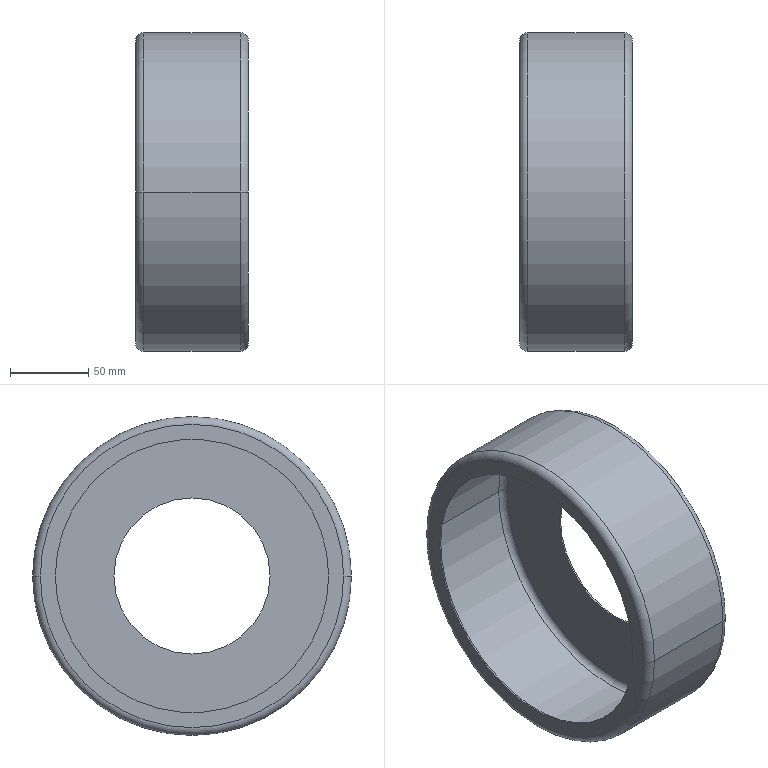Component | SolidWorks | Flywheel-1 | 1 solid | 20 faces | box 72.09 x 204.25 x 204.25 mm | volume 75898 mm3 | cylinder 8 | torus 8 | plane 4 | commonest cylinder face diameters 100 x2 204.252 x2 175 x2 202.252 x2
build123d program:
from build123d import *

# Parameters (mm, degrees)
SKETCH2_R                 = 50
REPAIR_CAMSHAFTHOLE_DEPTH = 1.75


with BuildPart() as part:
    # Sketch1 → Revolve1 (revolve)
    with BuildSketch(Plane(origin=(0, 0, 0), x_dir=(1, 0, 0), z_dir=(0, 1, 0))):
        with BuildLine():
            Line((97.126, 75), (0, 75))
            Line((0, 75), (0, 74))
            Line((0, 74), (97.126, 74))
            ThreePointArc((97.126, 74), (99.954, 72.828), (101.126, 70))
            Line((101.126, 70), (101.126, 7.905))
            ThreePointArc((101.126, 7.905), (99.954, 5.077), (97.126, 3.905))
            Line((97.126, 3.905), (87.5, 3.905))
            Line((87.5, 3.905), (87.5, 2.905))
            Line((87.5, 2.905), (97.126, 2.905))
            ThreePointArc((97.126, 2.905), (100.662, 4.37), (102.126, 7.905))
            Line((102.126, 7.905), (102.126, 70))
            ThreePointArc((102.126, 70), (100.662, 73.536), (97.126, 75))
        make_face()
    revolve(axis=Axis((0, 0, -75.001), (0, 0, 1)))

    # Sketch2 → Repair_CamshaftHole (cut, symmetric)
    with BuildSketch(Plane.XY.offset(-74.457)):
        Circle(SKETCH2_R)
    extrude(amount=REPAIR_CAMSHAFTHOLE_DEPTH, both=True, mode=Mode.SUBTRACT)


solid = part.part

# Placed as in the assembly
solid = solid.moved(Location((-829.707, 870.769, 1116.347), (0, -90, 0)))
STEP:
#1=CARTESIAN_POINT('',(-29.713,36.251,43.951));
#2=VERTEX_POINT('',#1);
#3=CARTESIAN_POINT('',(-29.713,32.314,43.951));
#4=VERTEX_POINT('',#3);
#5=CARTESIAN_POINT('',(-29.713,34.282,43.951));
#6=DIRECTION('',(1.,0.,0.));
#7=DIRECTION('',(0.,-1.,0.));
#8=AXIS2_PLACEMENT_3D('',#5,#6,#7);
#9=CIRCLE('',#8,1.969);
#10=EDGE_CURVE('',#2,#4,#9,.T.);
#11=ORIENTED_EDGE('',*,*,#10,.T.);
#12=CARTESIAN_POINT('',(-29.752,32.314,43.951));
#13=VERTEX_POINT('',#12);
#14=CARTESIAN_POINT('',(-29.665,32.314,43.951));
#15=DIRECTION('',(-1.,0.,0.));
#16=VECTOR('',#15,39.37);
#17=LINE('',#14,#16);
#18=EDGE_CURVE('',#4,#13,#17,.T.);
#19=ORIENTED_EDGE('',*,*,#18,.T.);
#20=CARTESIAN_POINT('',(-29.752,36.251,43.951));
#21=VERTEX_POINT('',#20);
#22=CARTESIAN_POINT('',(-29.752,34.282,43.951));
#23=DIRECTION('',(-1.,0.,0.));
#24=DIRECTION('',(0.,1.,0.));
#25=AXIS2_PLACEMENT_3D('',#22,#23,#24);
#26=CIRCLE('',#25,1.969);
#27=EDGE_CURVE('',#13,#21,#26,.T.);
#28=ORIENTED_EDGE('',*,*,#27,.T.);
#29=CARTESIAN_POINT('',(-29.665,36.251,43.951));
#30=DIRECTION('',(-1.,0.,0.));
#31=VECTOR('',#30,39.37);
#32=LINE('',#29,#31);
#33=EDGE_CURVE('',#2,#21,#32,.T.);
#34=ORIENTED_EDGE('',*,*,#33,.F.);
#35=EDGE_LOOP('',(#11,#19,#28,#34));
#36=FACE_OUTER_BOUND('',#35,.T.);
#37=CARTESIAN_POINT('',(-29.665,34.282,43.951));
#38=DIRECTION('',(-1.,0.,0.));
#39=DIRECTION('',(0.,1.,0.));
#40=AXIS2_PLACEMENT_3D('',#37,#38,#39);
#41=CYLINDRICAL_SURFACE('',#40,1.969);
#42=ADVANCED_FACE('',(#36),#41,.F.);
#43=CARTESIAN_POINT('',(-29.91,38.303,43.951));
#44=VERTEX_POINT('',#43);
#45=CARTESIAN_POINT('',(-29.91,30.262,43.951));
#46=VERTEX_POINT('',#45);
#47=CARTESIAN_POINT('',(-29.91,34.282,43.951));
#48=DIRECTION('',(-1.,0.,0.));
#49=DIRECTION('',(0.,1.,0.));
#50=AXIS2_PLACEMENT_3D('',#47,#48,#49);
#51=CIRCLE('',#50,4.021);
#52=EDGE_CURVE('',#44,#46,#51,.T.);
#53=ORIENTED_EDGE('',*,*,#52,.T.);
#54=CARTESIAN_POINT('',(-32.354,30.262,43.951));
#55=VERTEX_POINT('',#54);
#56=CARTESIAN_POINT('',(-29.713,30.262,43.951));
#57=DIRECTION('',(-1.,0.,0.));
#58=VECTOR('',#57,39.37);
#59=LINE('',#56,#58);
#60=EDGE_CURVE('',#46,#55,#59,.T.);
#61=ORIENTED_EDGE('',*,*,#60,.T.);
#62=CARTESIAN_POINT('',(-32.354,38.303,43.951));
#63=VERTEX_POINT('',#62);
#64=CARTESIAN_POINT('',(-32.354,34.282,43.951));
#65=DIRECTION('',(-1.,0.,0.));
#66=DIRECTION('',(0.,1.,0.));
#67=AXIS2_PLACEMENT_3D('',#64,#65,#66);
#68=CIRCLE('',#67,4.021);
#69=EDGE_CURVE('',#63,#55,#68,.T.);
#70=ORIENTED_EDGE('',*,*,#69,.F.);
#71=CARTESIAN_POINT('',(-29.713,38.303,43.951));
#72=DIRECTION('',(-1.,0.,0.));
#73=VECTOR('',#72,39.37);
#74=LINE('',#71,#73);
#75=EDGE_CURVE('',#44,#63,#74,.T.);
#76=ORIENTED_EDGE('',*,*,#75,.F.);
#77=EDGE_LOOP('',(#53,#61,#70,#76));
#78=FACE_OUTER_BOUND('',#77,.T.);
#79=CARTESIAN_POINT('',(-29.713,34.282,43.951));
#80=DIRECTION('',(-1.,0.,0.));
#81=DIRECTION('',(0.,1.,0.));
#82=AXIS2_PLACEMENT_3D('',#79,#80,#81);
#83=CYLINDRICAL_SURFACE('',#82,4.021);
#84=ADVANCED_FACE('',(#78),#83,.T.);
#85=ORIENTED_EDGE('',*,*,#69,.T.);
#86=CARTESIAN_POINT('',(-32.551,30.458,43.951));
#87=VERTEX_POINT('',#86);
#88=CARTESIAN_POINT('',(-32.354,30.458,43.951));
#89=DIRECTION('',(0.,0.,-1.));
#90=DIRECTION('',(0.,1.,0.));
#91=AXIS2_PLACEMENT_3D('',#88,#89,#90);
#92=CIRCLE('',#91,0.1969);
#93=EDGE_CURVE('',#55,#87,#92,.T.);
#94=ORIENTED_EDGE('',*,*,#93,.T.);
#95=CARTESIAN_POINT('',(-32.551,38.106,43.951));
#96=VERTEX_POINT('',#95);
#97=CARTESIAN_POINT('',(-32.551,34.282,43.951));
#98=DIRECTION('',(-1.,0.,0.));
#99=DIRECTION('',(0.,1.,0.));
#100=AXIS2_PLACEMENT_3D('',#97,#98,#99);
#101=CIRCLE('',#100,3.824);
#102=EDGE_CURVE('',#96,#87,#101,.T.);
#103=ORIENTED_EDGE('',*,*,#102,.F.);
#104=CARTESIAN_POINT('',(-32.354,38.106,43.951));
#105=DIRECTION('',(0.,0.,1.));
#106=DIRECTION('',(1.,0.,0.));
#107=AXIS2_PLACEMENT_3D('',#104,#105,#106);
#108=CIRCLE('',#107,0.1969);
#109=EDGE_CURVE('',#63,#96,#108,.T.);
#110=ORIENTED_EDGE('',*,*,#109,.F.);
#111=EDGE_LOOP('',(#85,#94,#103,#110));
#112=FACE_OUTER_BOUND('',#111,.T.);
#113=CARTESIAN_POINT('',(-32.354,34.282,43.951));
#114=DIRECTION('',(-1.,0.,0.));
#115=DIRECTION('',(0.,1.,0.));
#116=AXIS2_PLACEMENT_3D('',#113,#114,#115);
#117=TOROIDAL_SURFACE('',#116,3.824,0.1969);
#118=ADVANCED_FACE('',(#112),#117,.T.);
#119=CARTESIAN_POINT('',(-32.512,30.837,43.951));
#120=VERTEX_POINT('',#119);
#121=CARTESIAN_POINT('',(-32.512,37.727,43.951));
#122=VERTEX_POINT('',#121);
#123=CARTESIAN_POINT('',(-32.512,34.282,43.951));
#124=DIRECTION('',(-1.,0.,0.));
#125=DIRECTION('',(0.,1.,0.));
#126=AXIS2_PLACEMENT_3D('',#123,#124,#125);
#127=CIRCLE('',#126,3.445);
#128=EDGE_CURVE('',#120,#122,#127,.T.);
#129=ORIENTED_EDGE('',*,*,#128,.F.);
#130=CARTESIAN_POINT('',(-32.551,30.837,43.951));
#131=VERTEX_POINT('',#130);
#132=CARTESIAN_POINT('',(-29.713,30.837,43.951));
#133=DIRECTION('',(-1.,0.,0.));
#134=VECTOR('',#133,39.37);
#135=LINE('',#132,#134);
#136=EDGE_CURVE('',#120,#131,#135,.T.);
#137=ORIENTED_EDGE('',*,*,#136,.T.);
#138=CARTESIAN_POINT('',(-32.551,37.727,43.951));
#139=VERTEX_POINT('',#138);
#140=CARTESIAN_POINT('',(-32.551,34.282,43.951));
#141=DIRECTION('',(-1.,0.,0.));
#142=DIRECTION('',(0.,1.,0.));
#143=AXIS2_PLACEMENT_3D('',#140,#141,#142);
#144=CIRCLE('',#143,3.445);
#145=EDGE_CURVE('',#131,#139,#144,.T.);
#146=ORIENTED_EDGE('',*,*,#145,.T.);
#147=CARTESIAN_POINT('',(-29.713,37.727,43.951));
#148=DIRECTION('',(-1.,0.,0.));
#149=VECTOR('',#148,39.37);
#150=LINE('',#147,#149);
#151=EDGE_CURVE('',#122,#139,#150,.T.);
#152=ORIENTED_EDGE('',*,*,#151,.F.);
#153=EDGE_LOOP('',(#129,#137,#146,#152));
#154=FACE_OUTER_BOUND('',#153,.T.);
#155=CARTESIAN_POINT('',(-29.713,34.282,43.951));
#156=DIRECTION('',(-1.,0.,0.));
#157=DIRECTION('',(0.,1.,0.));
#158=AXIS2_PLACEMENT_3D('',#155,#156,#157);
#159=CYLINDRICAL_SURFACE('',#158,3.445);
#160=ADVANCED_FACE('',(#154),#159,.F.);
#161=CARTESIAN_POINT('',(-32.354,30.301,43.951));
#162=VERTEX_POINT('',#161);
#163=CARTESIAN_POINT('',(-32.354,38.264,43.951));
#164=VERTEX_POINT('',#163);
#165=CARTESIAN_POINT('',(-32.354,34.282,43.951));
#166=DIRECTION('',(-1.,0.,0.));
#167=DIRECTION('',(0.,1.,0.));
#168=AXIS2_PLACEMENT_3D('',#165,#166,#167);
#169=CIRCLE('',#168,3.981);
#170=EDGE_CURVE('',#162,#164,#169,.T.);
#171=ORIENTED_EDGE('',*,*,#170,.F.);
#172=CARTESIAN_POINT('',(-32.512,30.458,43.951));
#173=VERTEX_POINT('',#172);
#174=CARTESIAN_POINT('',(-32.354,30.458,43.951));
#175=DIRECTION('',(0.,0.,-1.));
#176=DIRECTION('',(0.,1.,0.));
#177=AXIS2_PLACEMENT_3D('',#174,#175,#176);
#178=CIRCLE('',#177,0.1575);
#179=EDGE_CURVE('',#162,#173,#178,.T.);
#180=ORIENTED_EDGE('',*,*,#179,.T.);
#181=CARTESIAN_POINT('',(-32.512,38.106,43.951));
#182=VERTEX_POINT('',#181);
#183=CARTESIAN_POINT('',(-32.512,34.282,43.951));
#184=DIRECTION('',(-1.,0.,0.));
#185=DIRECTION('',(0.,1.,0.));
#186=AXIS2_PLACEMENT_3D('',#183,#184,#185);
#187=CIRCLE('',#186,3.824);
#188=EDGE_CURVE('',#173,#182,#187,.T.);
#189=ORIENTED_EDGE('',*,*,#188,.T.);
#190=CARTESIAN_POINT('',(-32.354,38.106,43.951));
#191=DIRECTION('',(0.,0.,1.));
#192=DIRECTION('',(1.,0.,0.));
#193=AXIS2_PLACEMENT_3D('',#190,#191,#192);
#194=CIRCLE('',#193,0.1575);
#195=EDGE_CURVE('',#164,#182,#194,.T.);
#196=ORIENTED_EDGE('',*,*,#195,.F.);
#197=EDGE_LOOP('',(#171,#180,#189,#196));
#198=FACE_OUTER_BOUND('',#197,.T.);
#199=CARTESIAN_POINT('',(-32.354,34.282,43.951));
#200=DIRECTION('',(-1.,0.,0.));
#201=DIRECTION('',(0.,1.,0.));
#202=AXIS2_PLACEMENT_3D('',#199,#200,#201);
#203=TOROIDAL_SURFACE('',#202,3.824,0.1575);
#204=ADVANCED_FACE('',(#198),#203,.F.);
#205=CARTESIAN_POINT('',(-29.91,30.301,43.951));
#206=VERTEX_POINT('',#205);
#207=CARTESIAN_POINT('',(-29.91,38.264,43.951));
#208=VERTEX_POINT('',#207);
#209=CARTESIAN_POINT('',(-29.91,34.282,43.951));
#210=DIRECTION('',(-1.,0.,0.));
#211=DIRECTION('',(0.,1.,0.));
#212=AXIS2_PLACEMENT_3D('',#209,#210,#211);
#213=CIRCLE('',#212,3.981);
#214=EDGE_CURVE('',#206,#208,#213,.T.);
#215=ORIENTED_EDGE('',*,*,#214,.F.);
#216=CARTESIAN_POINT('',(-29.713,30.301,43.951));
#217=DIRECTION('',(-1.,0.,0.));
#218=VECTOR('',#217,39.37);
#219=LINE('',#216,#218);
#220=EDGE_CURVE('',#206,#162,#219,.T.);
#221=ORIENTED_EDGE('',*,*,#220,.T.);
#222=ORIENTED_EDGE('',*,*,#170,.T.);
#223=CARTESIAN_POINT('',(-29.713,38.264,43.951));
#224=DIRECTION('',(-1.,0.,0.));
#225=VECTOR('',#224,39.37);
#226=LINE('',#223,#225);
#227=EDGE_CURVE('',#208,#164,#226,.T.);
#228=ORIENTED_EDGE('',*,*,#227,.F.);
#229=EDGE_LOOP('',(#215,#221,#222,#228));
#230=FACE_OUTER_BOUND('',#229,.T.);
#231=CARTESIAN_POINT('',(-29.713,34.282,43.951));
#232=DIRECTION('',(-1.,0.,0.));
#233=DIRECTION('',(0.,1.,0.));
#234=AXIS2_PLACEMENT_3D('',#231,#232,#233);
#235=CYLINDRICAL_SURFACE('',#234,3.981);
#236=ADVANCED_FACE('',(#230),#235,.F.);
#237=CARTESIAN_POINT('',(-29.752,30.458,43.951));
#238=VERTEX_POINT('',#237);
#239=CARTESIAN_POINT('',(-29.752,38.106,43.951));
#240=VERTEX_POINT('',#239);
#241=CARTESIAN_POINT('',(-29.752,34.282,43.951));
#242=DIRECTION('',(-1.,0.,0.));
#243=DIRECTION('',(0.,1.,0.));
#244=AXIS2_PLACEMENT_3D('',#241,#242,#243);
#245=CIRCLE('',#244,3.824);
#246=EDGE_CURVE('',#238,#240,#245,.T.);
#247=ORIENTED_EDGE('',*,*,#246,.F.);
#248=CARTESIAN_POINT('',(-29.91,30.458,43.951));
#249=DIRECTION('',(0.,0.,-1.));
#250=DIRECTION('',(0.,1.,0.));
#251=AXIS2_PLACEMENT_3D('',#248,#249,#250);
#252=CIRCLE('',#251,0.1575);
#253=EDGE_CURVE('',#238,#206,#252,.T.);
#254=ORIENTED_EDGE('',*,*,#253,.T.);
#255=ORIENTED_EDGE('',*,*,#214,.T.);
#256=CARTESIAN_POINT('',(-29.91,38.106,43.951));
#257=DIRECTION('',(0.,0.,1.));
#258=DIRECTION('',(1.,0.,0.));
#259=AXIS2_PLACEMENT_3D('',#256,#257,#258);
#260=CIRCLE('',#259,0.1575);
#261=EDGE_CURVE('',#240,#208,#260,.T.);
#262=ORIENTED_EDGE('',*,*,#261,.F.);
#263=EDGE_LOOP('',(#247,#254,#255,#262));
#264=FACE_OUTER_BOUND('',#263,.T.);
#265=CARTESIAN_POINT('',(-29.91,34.282,43.951));
#266=DIRECTION('',(-1.,0.,0.));
#267=DIRECTION('',(0.,1.,0.));
#268=AXIS2_PLACEMENT_3D('',#265,#266,#267);
#269=TOROIDAL_SURFACE('',#268,3.824,0.1575);
#270=ADVANCED_FACE('',(#264),#269,.F.);
#271=CARTESIAN_POINT('',(-29.713,38.106,43.951));
#272=VERTEX_POINT('',#271);
#273=CARTESIAN_POINT('',(-29.713,30.458,43.951));
#274=VERTEX_POINT('',#273);
#275=CARTESIAN_POINT('',(-29.713,34.282,43.951));
#276=DIRECTION('',(-1.,0.,0.));
#277=DIRECTION('',(0.,1.,0.));
#278=AXIS2_PLACEMENT_3D('',#275,#276,#277);
#279=CIRCLE('',#278,3.824);
#280=EDGE_CURVE('',#272,#274,#279,.T.);
#281=ORIENTED_EDGE('',*,*,#280,.T.);
#282=CARTESIAN_POINT('',(-29.91,30.458,43.951));
#283=DIRECTION('',(0.,0.,-1.));
#284=DIRECTION('',(0.,1.,0.));
#285=AXIS2_PLACEMENT_3D('',#282,#283,#284);
#286=CIRCLE('',#285,0.1969);
#287=EDGE_CURVE('',#274,#46,#286,.T.);
#288=ORIENTED_EDGE('',*,*,#287,.T.);
#289=ORIENTED_EDGE('',*,*,#52,.F.);
#290=CARTESIAN_POINT('',(-29.91,38.106,43.951));
#291=DIRECTION('',(0.,0.,1.));
#292=DIRECTION('',(1.,0.,0.));
#293=AXIS2_PLACEMENT_3D('',#290,#291,#292);
#294=CIRCLE('',#293,0.1969);
#295=EDGE_CURVE('',#272,#44,#294,.T.);
#296=ORIENTED_EDGE('',*,*,#295,.F.);
#297=EDGE_LOOP('',(#281,#288,#289,#296));
#298=FACE_OUTER_BOUND('',#297,.T.);
#299=CARTESIAN_POINT('',(-29.91,34.282,43.951));
#300=DIRECTION('',(-1.,0.,0.));
#301=DIRECTION('',(0.,1.,0.));
#302=AXIS2_PLACEMENT_3D('',#299,#300,#301);
#303=TOROIDAL_SURFACE('',#302,3.824,0.1969);
#304=ADVANCED_FACE('',(#298),#303,.T.);
#305=ORIENTED_EDGE('',*,*,#287,.F.);
#306=CARTESIAN_POINT('',(-29.713,34.282,43.951));
#307=DIRECTION('',(-1.,0.,0.));
#308=DIRECTION('',(0.,1.,0.));
#309=AXIS2_PLACEMENT_3D('',#306,#307,#308);
#310=CIRCLE('',#309,3.824);
#311=EDGE_CURVE('',#274,#272,#310,.T.);
#312=ORIENTED_EDGE('',*,*,#311,.T.);
#313=ORIENTED_EDGE('',*,*,#295,.T.);
#314=CARTESIAN_POINT('',(-29.91,34.282,43.951));
#315=DIRECTION('',(-1.,0.,0.));
#316=DIRECTION('',(0.,1.,0.));
#317=AXIS2_PLACEMENT_3D('',#314,#315,#316);
#318=CIRCLE('',#317,4.021);
#319=EDGE_CURVE('',#46,#44,#318,.T.);
#320=ORIENTED_EDGE('',*,*,#319,.F.);
#321=EDGE_LOOP('',(#305,#312,#313,#320));
#322=FACE_OUTER_BOUND('',#321,.T.);
#323=CARTESIAN_POINT('',(-29.91,34.282,43.951));
#324=DIRECTION('',(-1.,0.,0.));
#325=DIRECTION('',(0.,1.,0.));
#326=AXIS2_PLACEMENT_3D('',#323,#324,#325);
#327=TOROIDAL_SURFACE('',#326,3.824,0.1969);
#328=ADVANCED_FACE('',(#322),#327,.T.);
#329=ORIENTED_EDGE('',*,*,#10,.F.);
#330=CARTESIAN_POINT('',(-29.713,34.282,43.951));
#331=DIRECTION('',(1.,0.,0.));
#332=DIRECTION('',(0.,-1.,0.));
#333=AXIS2_PLACEMENT_3D('',#330,#331,#332);
#334=CIRCLE('',#333,1.969);
#335=EDGE_CURVE('',#4,#2,#334,.T.);
#336=ORIENTED_EDGE('',*,*,#335,.F.);
#337=EDGE_LOOP('',(#329,#336));
#338=FACE_BOUND('',#337,.T.);
#339=ORIENTED_EDGE('',*,*,#280,.F.);
#340=ORIENTED_EDGE('',*,*,#311,.F.);
#341=EDGE_LOOP('',(#339,#340));
#342=FACE_OUTER_BOUND('',#341,.T.);
#343=CARTESIAN_POINT('',(-29.713,38.106,43.951));
#344=DIRECTION('',(1.,0.,0.));
#345=DIRECTION('',(0.,-1.,0.));
#346=AXIS2_PLACEMENT_3D('',#343,#344,#345);
#347=PLANE('',#346);
#348=ADVANCED_FACE('',(#338,#342),#347,.T.);
#349=CARTESIAN_POINT('',(-29.752,34.282,43.951));
#350=DIRECTION('',(-1.,0.,0.));
#351=DIRECTION('',(0.,1.,0.));
#352=AXIS2_PLACEMENT_3D('',#349,#350,#351);
#353=CIRCLE('',#352,1.969);
#354=EDGE_CURVE('',#21,#13,#353,.T.);
#355=ORIENTED_EDGE('',*,*,#354,.F.);
#356=ORIENTED_EDGE('',*,*,#27,.F.);
#357=EDGE_LOOP('',(#355,#356));
#358=FACE_BOUND('',#357,.T.);
#359=CARTESIAN_POINT('',(-29.752,34.282,43.951));
#360=DIRECTION('',(-1.,0.,0.));
#361=DIRECTION('',(0.,1.,0.));
#362=AXIS2_PLACEMENT_3D('',#359,#360,#361);
#363=CIRCLE('',#362,3.824);
#364=EDGE_CURVE('',#240,#238,#363,.T.);
#365=ORIENTED_EDGE('',*,*,#364,.T.);
#366=ORIENTED_EDGE('',*,*,#246,.T.);
#367=EDGE_LOOP('',(#365,#366));
#368=FACE_OUTER_BOUND('',#367,.T.);
#369=CARTESIAN_POINT('',(-29.752,34.282,43.951));
#370=DIRECTION('',(-1.,0.,0.));
#371=DIRECTION('',(0.,1.,0.));
#372=AXIS2_PLACEMENT_3D('',#369,#370,#371);
#373=PLANE('',#372);
#374=ADVANCED_FACE('',(#358,#368),#373,.T.);
#375=ORIENTED_EDGE('',*,*,#253,.F.);
#376=ORIENTED_EDGE('',*,*,#364,.F.);
#377=ORIENTED_EDGE('',*,*,#261,.T.);
#378=CARTESIAN_POINT('',(-29.91,34.282,43.951));
#379=DIRECTION('',(-1.,0.,0.));
#380=DIRECTION('',(0.,1.,0.));
#381=AXIS2_PLACEMENT_3D('',#378,#379,#380);
#382=CIRCLE('',#381,3.981);
#383=EDGE_CURVE('',#208,#206,#382,.T.);
#384=ORIENTED_EDGE('',*,*,#383,.T.);
#385=EDGE_LOOP('',(#375,#376,#377,#384));
#386=FACE_OUTER_BOUND('',#385,.T.);
#387=CARTESIAN_POINT('',(-29.91,34.282,43.951));
#388=DIRECTION('',(-1.,0.,0.));
#389=DIRECTION('',(0.,1.,0.));
#390=AXIS2_PLACEMENT_3D('',#387,#388,#389);
#391=TOROIDAL_SURFACE('',#390,3.824,0.1575);
#392=ADVANCED_FACE('',(#386),#391,.F.);
#393=ORIENTED_EDGE('',*,*,#220,.F.);
#394=ORIENTED_EDGE('',*,*,#383,.F.);
#395=ORIENTED_EDGE('',*,*,#227,.T.);
#396=CARTESIAN_POINT('',(-32.354,34.282,43.951));
#397=DIRECTION('',(-1.,0.,0.));
#398=DIRECTION('',(0.,1.,0.));
#399=AXIS2_PLACEMENT_3D('',#396,#397,#398);
#400=CIRCLE('',#399,3.981);
#401=EDGE_CURVE('',#164,#162,#400,.T.);
#402=ORIENTED_EDGE('',*,*,#401,.T.);
#403=EDGE_LOOP('',(#393,#394,#395,#402));
#404=FACE_OUTER_BOUND('',#403,.T.);
#405=CARTESIAN_POINT('',(-29.713,34.282,43.951));
#406=DIRECTION('',(-1.,0.,0.));
#407=DIRECTION('',(0.,1.,0.));
#408=AXIS2_PLACEMENT_3D('',#405,#406,#407);
#409=CYLINDRICAL_SURFACE('',#408,3.981);
#410=ADVANCED_FACE('',(#404),#409,.F.);
#411=ORIENTED_EDGE('',*,*,#179,.F.);
#412=ORIENTED_EDGE('',*,*,#401,.F.);
#413=ORIENTED_EDGE('',*,*,#195,.T.);
#414=CARTESIAN_POINT('',(-32.512,34.282,43.951));
#415=DIRECTION('',(-1.,0.,0.));
#416=DIRECTION('',(0.,1.,0.));
#417=AXIS2_PLACEMENT_3D('',#414,#415,#416);
#418=CIRCLE('',#417,3.824);
#419=EDGE_CURVE('',#182,#173,#418,.T.);
#420=ORIENTED_EDGE('',*,*,#419,.T.);
#421=EDGE_LOOP('',(#411,#412,#413,#420));
#422=FACE_OUTER_BOUND('',#421,.T.);
#423=CARTESIAN_POINT('',(-32.354,34.282,43.951));
#424=DIRECTION('',(-1.,0.,0.));
#425=DIRECTION('',(0.,1.,0.));
#426=AXIS2_PLACEMENT_3D('',#423,#424,#425);
#427=TOROIDAL_SURFACE('',#426,3.824,0.1575);
#428=ADVANCED_FACE('',(#422),#427,.F.);
#429=CARTESIAN_POINT('',(-32.512,34.282,43.951));
#430=DIRECTION('',(-1.,0.,0.));
#431=DIRECTION('',(0.,1.,0.));
#432=AXIS2_PLACEMENT_3D('',#429,#430,#431);
#433=CIRCLE('',#432,3.445);
#434=EDGE_CURVE('',#122,#120,#433,.T.);
#435=ORIENTED_EDGE('',*,*,#434,.T.);
#436=ORIENTED_EDGE('',*,*,#128,.T.);
#437=EDGE_LOOP('',(#435,#436));
#438=FACE_BOUND('',#437,.T.);
#439=ORIENTED_EDGE('',*,*,#419,.F.);
#440=ORIENTED_EDGE('',*,*,#188,.F.);
#441=EDGE_LOOP('',(#439,#440));
#442=FACE_OUTER_BOUND('',#441,.T.);
#443=CARTESIAN_POINT('',(-32.512,38.106,43.951));
#444=DIRECTION('',(1.,0.,0.));
#445=DIRECTION('',(0.,-1.,0.));
#446=AXIS2_PLACEMENT_3D('',#443,#444,#445);
#447=PLANE('',#446);
#448=ADVANCED_FACE('',(#438,#442),#447,.T.);
#449=ORIENTED_EDGE('',*,*,#136,.F.);
#450=ORIENTED_EDGE('',*,*,#434,.F.);
#451=ORIENTED_EDGE('',*,*,#151,.T.);
#452=CARTESIAN_POINT('',(-32.551,34.282,43.951));
#453=DIRECTION('',(-1.,0.,0.));
#454=DIRECTION('',(0.,1.,0.));
#455=AXIS2_PLACEMENT_3D('',#452,#453,#454);
#456=CIRCLE('',#455,3.445);
#457=EDGE_CURVE('',#139,#131,#456,.T.);
#458=ORIENTED_EDGE('',*,*,#457,.T.);
#459=EDGE_LOOP('',(#449,#450,#451,#458));
#460=FACE_OUTER_BOUND('',#459,.T.);
#461=CARTESIAN_POINT('',(-29.713,34.282,43.951));
#462=DIRECTION('',(-1.,0.,0.));
#463=DIRECTION('',(0.,1.,0.));
#464=AXIS2_PLACEMENT_3D('',#461,#462,#463);
#465=CYLINDRICAL_SURFACE('',#464,3.445);
#466=ADVANCED_FACE('',(#460),#465,.F.);
#467=ORIENTED_EDGE('',*,*,#102,.T.);
#468=CARTESIAN_POINT('',(-32.551,34.282,43.951));
#469=DIRECTION('',(-1.,0.,0.));
#470=DIRECTION('',(0.,1.,0.));
#471=AXIS2_PLACEMENT_3D('',#468,#469,#470);
#472=CIRCLE('',#471,3.824);
#473=EDGE_CURVE('',#87,#96,#472,.T.);
#474=ORIENTED_EDGE('',*,*,#473,.T.);
#475=EDGE_LOOP('',(#467,#474));
#476=FACE_OUTER_BOUND('',#475,.T.);
#477=ORIENTED_EDGE('',*,*,#457,.F.);
#478=ORIENTED_EDGE('',*,*,#145,.F.);
#479=EDGE_LOOP('',(#477,#478));
#480=FACE_BOUND('',#479,.T.);
#481=CARTESIAN_POINT('',(-32.551,37.727,43.951));
#482=DIRECTION('',(-1.,0.,0.));
#483=DIRECTION('',(0.,1.,0.));
#484=AXIS2_PLACEMENT_3D('',#481,#482,#483);
#485=PLANE('',#484);
#486=ADVANCED_FACE('',(#476,#480),#485,.T.);
#487=ORIENTED_EDGE('',*,*,#93,.F.);
#488=CARTESIAN_POINT('',(-32.354,34.282,43.951));
#489=DIRECTION('',(-1.,0.,0.));
#490=DIRECTION('',(0.,1.,0.));
#491=AXIS2_PLACEMENT_3D('',#488,#489,#490);
#492=CIRCLE('',#491,4.021);
#493=EDGE_CURVE('',#55,#63,#492,.T.);
#494=ORIENTED_EDGE('',*,*,#493,.T.);
#495=ORIENTED_EDGE('',*,*,#109,.T.);
#496=ORIENTED_EDGE('',*,*,#473,.F.);
#497=EDGE_LOOP('',(#487,#494,#495,#496));
#498=FACE_OUTER_BOUND('',#497,.T.);
#499=CARTESIAN_POINT('',(-32.354,34.282,43.951));
#500=DIRECTION('',(-1.,0.,0.));
#501=DIRECTION('',(0.,1.,0.));
#502=AXIS2_PLACEMENT_3D('',#499,#500,#501);
#503=TOROIDAL_SURFACE('',#502,3.824,0.1969);
#504=ADVANCED_FACE('',(#498),#503,.T.);
#505=ORIENTED_EDGE('',*,*,#60,.F.);
#506=ORIENTED_EDGE('',*,*,#319,.T.);
#507=ORIENTED_EDGE('',*,*,#75,.T.);
#508=ORIENTED_EDGE('',*,*,#493,.F.);
#509=EDGE_LOOP('',(#505,#506,#507,#508));
#510=FACE_OUTER_BOUND('',#509,.T.);
#511=CARTESIAN_POINT('',(-29.713,34.282,43.951));
#512=DIRECTION('',(-1.,0.,0.));
#513=DIRECTION('',(0.,1.,0.));
#514=AXIS2_PLACEMENT_3D('',#511,#512,#513);
#515=CYLINDRICAL_SURFACE('',#514,4.021);
#516=ADVANCED_FACE('',(#510),#515,.T.);
#517=ORIENTED_EDGE('',*,*,#18,.F.);
#518=ORIENTED_EDGE('',*,*,#335,.T.);
#519=ORIENTED_EDGE('',*,*,#33,.T.);
#520=ORIENTED_EDGE('',*,*,#354,.T.);
#521=EDGE_LOOP('',(#517,#518,#519,#520));
#522=FACE_OUTER_BOUND('',#521,.T.);
#523=CARTESIAN_POINT('',(-29.665,34.282,43.951));
#524=DIRECTION('',(-1.,0.,0.));
#525=DIRECTION('',(0.,1.,0.));
#526=AXIS2_PLACEMENT_3D('',#523,#524,#525);
#527=CYLINDRICAL_SURFACE('',#526,1.969);
#528=ADVANCED_FACE('',(#522),#527,.F.);
#529=CLOSED_SHELL('',(#42,#84,#118,#160,#204,#236,#270,#304,#328,#348,#374,#392,#410,#428,#448,#466,#486,#504,#516,#528));
#530=MANIFOLD_SOLID_BREP('',#529);
#531=CARTESIAN_POINT('',(0.,0.,0.));
#532=DIRECTION('',(0.,0.,1.));
#533=DIRECTION('',(1.,0.,0.));
#534=AXIS2_PLACEMENT_3D('',#531,#532,#533);
#535=(LENGTH_UNIT()NAMED_UNIT(*)SI_UNIT($,.METRE.));
#536=LENGTH_MEASURE_WITH_UNIT(LENGTH_MEASURE(0.0254),#535);
#537=DIMENSIONAL_EXPONENTS(1.,0.,0.,0.,0.,0.,0.);
#538=(CONVERSION_BASED_UNIT('',#536)LENGTH_UNIT()NAMED_UNIT(#537));
#539=UNCERTAINTY_MEASURE_WITH_UNIT(LENGTH_MEASURE(0.00001),#538,'','');
#540=(NAMED_UNIT(*)PLANE_ANGLE_UNIT()SI_UNIT($,.RADIAN.));
#541=(NAMED_UNIT(*)SI_UNIT($,.STERADIAN.)SOLID_ANGLE_UNIT());
#542=(GEOMETRIC_REPRESENTATION_CONTEXT(3)GLOBAL_UNCERTAINTY_ASSIGNED_CONTEXT((#539))GLOBAL_UNIT_ASSIGNED_CONTEXT((#538,#540,#541))REPRESENTATION_CONTEXT('',''));
#543=ADVANCED_BREP_SHAPE_REPRESENTATION('',(#530,#534),#542);
#544=COLOUR_RGB('',0.7922,0.8196,0.9333);
#545=FILL_AREA_STYLE_COLOUR('',#544);
#546=FILL_AREA_STYLE('',(#545));
#547=SURFACE_STYLE_FILL_AREA(#546);
#548=SURFACE_SIDE_STYLE('',(#547));
#549=SURFACE_STYLE_USAGE(.BOTH.,#548);
#550=PRESENTATION_STYLE_ASSIGNMENT((#549));
#551=STYLED_ITEM('',(#550),#530);
#552=PRESENTATION_LAYER_ASSIGNMENT('','',(#551));
#553=(LENGTH_UNIT()NAMED_UNIT(*)SI_UNIT($,.METRE.));
#554=LENGTH_MEASURE_WITH_UNIT(LENGTH_MEASURE(0.0254),#553);
#555=DIMENSIONAL_EXPONENTS(1.,0.,0.,0.,0.,0.,0.);
#556=(CONVERSION_BASED_UNIT('',#554)LENGTH_UNIT()NAMED_UNIT(#555));
#557=UNCERTAINTY_MEASURE_WITH_UNIT(LENGTH_MEASURE(0.00001),#556,'','');
#558=(NAMED_UNIT(*)PLANE_ANGLE_UNIT()SI_UNIT($,.RADIAN.));
#559=(NAMED_UNIT(*)SI_UNIT($,.STERADIAN.)SOLID_ANGLE_UNIT());
#560=(GEOMETRIC_REPRESENTATION_CONTEXT(3)GLOBAL_UNCERTAINTY_ASSIGNED_CONTEXT((#557))GLOBAL_UNIT_ASSIGNED_CONTEXT((#556,#558,#559))REPRESENTATION_CONTEXT('',''));
#561=MECHANICAL_DESIGN_GEOMETRIC_PRESENTATION_REPRESENTATION('',(#551),#560);